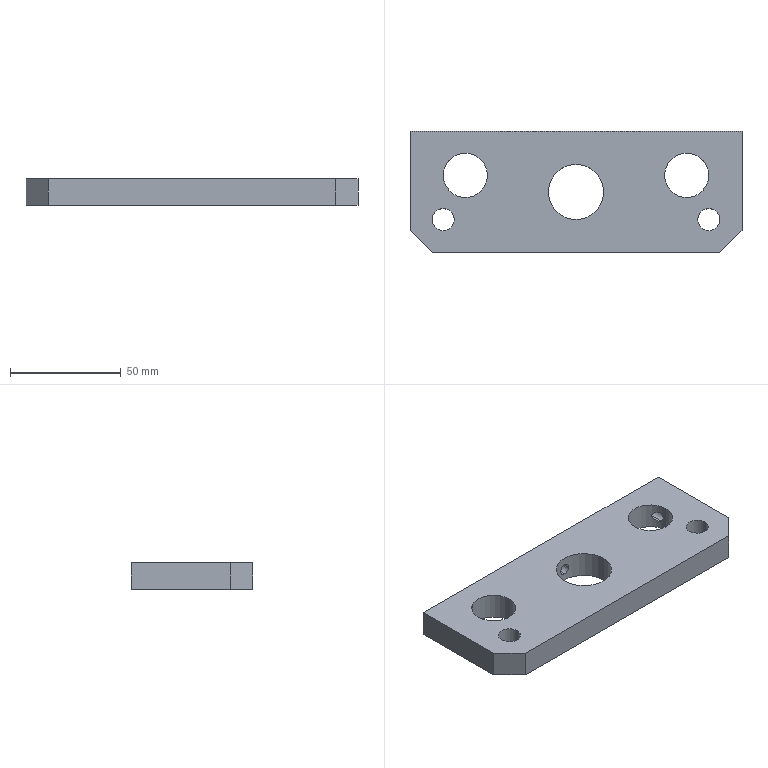Component | SolidWorks | ZTDJ-01-20-AxisMountingPlate-1 | 1 solid | 28 faces | box 150 x 55 x 12 mm | volume 81537 mm3 | cylinder 16 | plane 8 | cone 4 | commonest cylinder face diameters 5 x6 20 x4 10 x4 25 x2 | material 1023 Carbon Steel Sheet (SS)
build123d program:
from build123d import *

# Parameters (mm, degrees)
SKETCH1_W             = 150
SKETCH1_H             = 55
BOSS_EXTRUDE1_DEPTH   = 6
CHAMFER1_SIZE         = 10
M6_TAPPED_HOLE1_D     = 5
M6_TAPPED_HOLE1_DEPTH = 17
M6_TAPPED_HOLE1_TIP   = 1.502
SKETCH4_R             = 5
CUT_EXTRUDE1_DEPTH    = 81.779
SKETCH5_R             = 12.5
CUT_EXTRUDE2_DEPTH    = 81.779
SKETCH6_R             = 10
CUT_EXTRUDE3_DEPTH    = 81.779


with BuildPart() as part:
    # Sketch1 → Boss-Extrude1 (new, symmetric)
    with BuildSketch(Plane.XY):
        Rectangle(SKETCH1_W, SKETCH1_H)
    extrude(amount=BOSS_EXTRUDE1_DEPTH, both=True)

    # Chamfer1
    chamfer1_edges = [part.edges().sort_by_distance(p)[0] for p in [
        (75, -27.5, 0),
        (-75, -27.5, 0),
    ]]
    chamfer(chamfer1_edges, length=CHAMFER1_SIZE)

    # M6 Tapped Hole1
    with Locations(Plane(origin=(0, 27.5, 0), x_dir=(1, 0, 0), z_dir=(0, 1, 0))):
        with Locations((0, 0), (-60, 0), (60, 0)):
            Hole(M6_TAPPED_HOLE1_D / 2, depth=M6_TAPPED_HOLE1_DEPTH)
            with Locations((0, 0, -(M6_TAPPED_HOLE1_DEPTH + M6_TAPPED_HOLE1_TIP / 2))):  # 118° drill point
                Cone(0, M6_TAPPED_HOLE1_D / 2, M6_TAPPED_HOLE1_TIP, mode=Mode.SUBTRACT)

    # Sketch4 → Cut-Extrude1 (cut, through all)
    with BuildSketch(Plane.XY.offset(6)):
        with Locations((-60, -12.5)):
            Circle(SKETCH4_R)
        with Locations(Location((60, -12.5, 0), (0, 0, 180))):
            Circle(SKETCH4_R)
    extrude(amount=-CUT_EXTRUDE1_DEPTH, mode=Mode.SUBTRACT)

    # Sketch5 → Cut-Extrude2 (cut, through all)
    with BuildSketch(Plane.XY.offset(6)):
        Circle(SKETCH5_R)
    extrude(amount=-CUT_EXTRUDE2_DEPTH, mode=Mode.SUBTRACT)

    # Sketch6 → Cut-Extrude3 (cut, through all)
    with BuildSketch(Plane.XY.offset(6)):
        with Locations((-50, 7.5)):
            Circle(SKETCH6_R)
        with Locations(Location((50, 7.5, 0), (0, 0, 180))):
            Circle(SKETCH6_R)
    extrude(amount=-CUT_EXTRUDE3_DEPTH, mode=Mode.SUBTRACT)


solid = part.part

# Placed as in the assembly
solid = solid.moved(Location((-28.439, -71.686, 324), (0, 0, 0)))